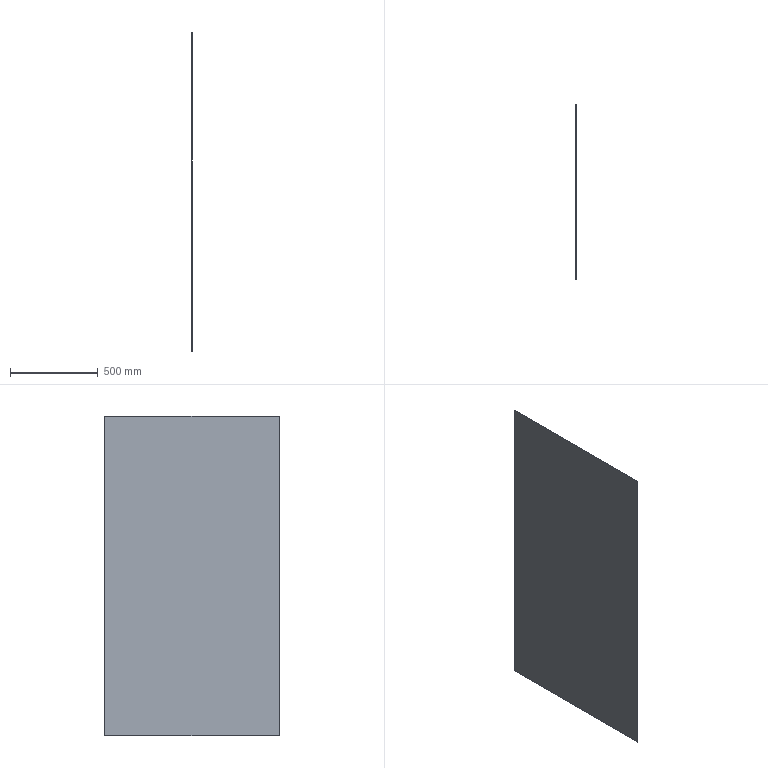Component | SolidWorks | BackPlate-3 | 1 solid | 9 faces | box 1.5 x 997 x 1820 mm | volume 2719006 mm3 | plane 9
STEP:
#1=COLOUR_RGB('',0.7922,0.8196,0.9333);
#2=FILL_AREA_STYLE_COLOUR('',#1);
#3=FILL_AREA_STYLE('',(#2));
#4=SURFACE_STYLE_FILL_AREA(#3);
#5=SURFACE_SIDE_STYLE('',(#4));
#6=SURFACE_STYLE_USAGE(.BOTH.,#5);
#7=PRESENTATION_STYLE_ASSIGNMENT((#6));
#8=CARTESIAN_POINT('',(19.524,29.311,66.594));
#9=VERTEX_POINT('',#8);
#10=CARTESIAN_POINT('',(19.508,29.311,66.594));
#11=VERTEX_POINT('',#10);
#12=CARTESIAN_POINT('',(19.567,29.311,66.594));
#13=DIRECTION('',(-1.,0.,0.));
#14=VECTOR('',#13,39.37);
#15=LINE('',#12,#14);
#16=EDGE_CURVE('',#9,#11,#15,.T.);
#17=ORIENTED_EDGE('',*,*,#16,.F.);
#18=CARTESIAN_POINT('',(19.524,29.311,-5.059));
#19=VERTEX_POINT('',#18);
#20=CARTESIAN_POINT('',(19.524,29.311,-5.059));
#21=DIRECTION('',(0.,0.,-1.));
#22=VECTOR('',#21,39.37);
#23=LINE('',#20,#22);
#24=EDGE_CURVE('',#9,#19,#23,.T.);
#25=ORIENTED_EDGE('',*,*,#24,.T.);
#26=CARTESIAN_POINT('',(19.508,29.311,-5.059));
#27=VERTEX_POINT('',#26);
#28=CARTESIAN_POINT('',(19.567,29.311,-5.059));
#29=DIRECTION('',(-1.,0.,0.));
#30=VECTOR('',#29,39.37);
#31=LINE('',#28,#30);
#32=EDGE_CURVE('',#19,#27,#31,.T.);
#33=ORIENTED_EDGE('',*,*,#32,.T.);
#34=CARTESIAN_POINT('',(19.508,29.311,-5.059));
#35=DIRECTION('',(0.,0.,-1.));
#36=VECTOR('',#35,39.37);
#37=LINE('',#34,#36);
#38=EDGE_CURVE('',#11,#27,#37,.T.);
#39=ORIENTED_EDGE('',*,*,#38,.F.);
#40=EDGE_LOOP('',(#17,#25,#33,#39));
#41=FACE_OUTER_BOUND('',#40,.T.);
#42=CARTESIAN_POINT('',(19.567,29.311,-5.059));
#43=DIRECTION('',(0.,1.,0.));
#44=DIRECTION('',(0.,0.,-1.));
#45=AXIS2_PLACEMENT_3D('',#42,#43,#44);
#46=PLANE('',#45);
#47=ADVANCED_FACE('',(#41),#46,.T.);
#48=CARTESIAN_POINT('',(19.524,-9.941,66.594));
#49=VERTEX_POINT('',#48);
#50=CARTESIAN_POINT('',(19.508,-9.941,66.594));
#51=VERTEX_POINT('',#50);
#52=CARTESIAN_POINT('',(19.567,-9.941,66.594));
#53=DIRECTION('',(-1.,0.,0.));
#54=VECTOR('',#53,39.37);
#55=LINE('',#52,#54);
#56=EDGE_CURVE('',#49,#51,#55,.T.);
#57=ORIENTED_EDGE('',*,*,#56,.F.);
#58=CARTESIAN_POINT('',(19.524,29.311,66.594));
#59=DIRECTION('',(0.,1.,0.));
#60=VECTOR('',#59,39.37);
#61=LINE('',#58,#60);
#62=EDGE_CURVE('',#49,#9,#61,.T.);
#63=ORIENTED_EDGE('',*,*,#62,.T.);
#64=ORIENTED_EDGE('',*,*,#16,.T.);
#65=CARTESIAN_POINT('',(19.508,-9.941,66.594));
#66=DIRECTION('',(0.,1.,0.));
#67=VECTOR('',#66,39.37);
#68=LINE('',#65,#67);
#69=EDGE_CURVE('',#51,#11,#68,.T.);
#70=ORIENTED_EDGE('',*,*,#69,.F.);
#71=EDGE_LOOP('',(#57,#63,#64,#70));
#72=FACE_OUTER_BOUND('',#71,.T.);
#73=CARTESIAN_POINT('',(19.567,-9.941,66.594));
#74=DIRECTION('',(0.,-0.,1.));
#75=DIRECTION('',(1.,-0.,-0.));
#76=AXIS2_PLACEMENT_3D('',#73,#74,#75);
#77=PLANE('',#76);
#78=ADVANCED_FACE('',(#72),#77,.T.);
#79=CARTESIAN_POINT('',(19.524,-9.941,-5.059));
#80=VERTEX_POINT('',#79);
#81=CARTESIAN_POINT('',(19.508,-9.941,-5.059));
#82=VERTEX_POINT('',#81);
#83=CARTESIAN_POINT('',(19.567,-9.941,-5.059));
#84=DIRECTION('',(-1.,0.,0.));
#85=VECTOR('',#84,39.37);
#86=LINE('',#83,#85);
#87=EDGE_CURVE('',#80,#82,#86,.T.);
#88=ORIENTED_EDGE('',*,*,#87,.F.);
#89=CARTESIAN_POINT('',(19.524,-9.941,66.594));
#90=DIRECTION('',(-0.,-0.,1.));
#91=VECTOR('',#90,39.37);
#92=LINE('',#89,#91);
#93=EDGE_CURVE('',#80,#49,#92,.T.);
#94=ORIENTED_EDGE('',*,*,#93,.T.);
#95=ORIENTED_EDGE('',*,*,#56,.T.);
#96=CARTESIAN_POINT('',(19.508,-9.941,-5.059));
#97=DIRECTION('',(-0.,-0.,1.));
#98=VECTOR('',#97,39.37);
#99=LINE('',#96,#98);
#100=EDGE_CURVE('',#82,#51,#99,.T.);
#101=ORIENTED_EDGE('',*,*,#100,.F.);
#102=EDGE_LOOP('',(#88,#94,#95,#101));
#103=FACE_OUTER_BOUND('',#102,.T.);
#104=CARTESIAN_POINT('',(19.567,-9.941,-5.059));
#105=DIRECTION('',(-0.,-1.,-0.));
#106=DIRECTION('',(-0.,-0.,1.));
#107=AXIS2_PLACEMENT_3D('',#104,#105,#106);
#108=PLANE('',#107);
#109=ADVANCED_FACE('',(#103),#108,.T.);
#110=ORIENTED_EDGE('',*,*,#32,.F.);
#111=CARTESIAN_POINT('',(19.567,29.268,-5.059));
#112=VERTEX_POINT('',#111);
#113=CARTESIAN_POINT('',(39.171,9.663,-5.059));
#114=DIRECTION('',(0.7071,-0.7071,-0.));
#115=VECTOR('',#114,39.37);
#116=LINE('',#113,#115);
#117=EDGE_CURVE('',#19,#112,#116,.T.);
#118=ORIENTED_EDGE('',*,*,#117,.T.);
#119=CARTESIAN_POINT('',(19.567,-9.898,-5.059));
#120=VERTEX_POINT('',#119);
#121=CARTESIAN_POINT('',(19.567,-9.941,-5.059));
#122=DIRECTION('',(-0.,-1.,-0.));
#123=VECTOR('',#122,39.37);
#124=LINE('',#121,#123);
#125=EDGE_CURVE('',#112,#120,#124,.T.);
#126=ORIENTED_EDGE('',*,*,#125,.T.);
#127=CARTESIAN_POINT('',(19.545,-9.919,-5.059));
#128=DIRECTION('',(-0.7071,-0.7071,-0.));
#129=VECTOR('',#128,39.37);
#130=LINE('',#127,#129);
#131=EDGE_CURVE('',#120,#80,#130,.T.);
#132=ORIENTED_EDGE('',*,*,#131,.T.);
#133=ORIENTED_EDGE('',*,*,#87,.T.);
#134=CARTESIAN_POINT('',(19.508,-9.941,-5.059));
#135=DIRECTION('',(-0.,-1.,-0.));
#136=VECTOR('',#135,39.37);
#137=LINE('',#134,#136);
#138=EDGE_CURVE('',#27,#82,#137,.T.);
#139=ORIENTED_EDGE('',*,*,#138,.F.);
#140=EDGE_LOOP('',(#110,#118,#126,#132,#133,#139));
#141=FACE_OUTER_BOUND('',#140,.T.);
#142=CARTESIAN_POINT('',(19.567,-9.941,-5.059));
#143=DIRECTION('',(-0.,0.,-1.));
#144=DIRECTION('',(-1.,0.,0.));
#145=AXIS2_PLACEMENT_3D('',#142,#143,#144);
#146=PLANE('',#145);
#147=ADVANCED_FACE('',(#141),#146,.T.);
#148=ORIENTED_EDGE('',*,*,#125,.F.);
#149=CARTESIAN_POINT('',(19.567,29.268,66.551));
#150=VERTEX_POINT('',#149);
#151=CARTESIAN_POINT('',(19.567,29.268,66.594));
#152=DIRECTION('',(-0.,-0.,1.));
#153=VECTOR('',#152,39.37);
#154=LINE('',#151,#153);
#155=EDGE_CURVE('',#112,#150,#154,.T.);
#156=ORIENTED_EDGE('',*,*,#155,.T.);
#157=CARTESIAN_POINT('',(19.567,-9.898,66.551));
#158=VERTEX_POINT('',#157);
#159=CARTESIAN_POINT('',(19.567,-9.941,66.551));
#160=DIRECTION('',(-0.,-1.,-0.));
#161=VECTOR('',#160,39.37);
#162=LINE('',#159,#161);
#163=EDGE_CURVE('',#150,#158,#162,.T.);
#164=ORIENTED_EDGE('',*,*,#163,.T.);
#165=CARTESIAN_POINT('',(19.567,-9.898,-5.059));
#166=DIRECTION('',(0.,0.,-1.));
#167=VECTOR('',#166,39.37);
#168=LINE('',#165,#167);
#169=EDGE_CURVE('',#158,#120,#168,.T.);
#170=ORIENTED_EDGE('',*,*,#169,.T.);
#171=EDGE_LOOP('',(#148,#156,#164,#170));
#172=FACE_OUTER_BOUND('',#171,.T.);
#173=CARTESIAN_POINT('',(19.567,9.685,30.768));
#174=DIRECTION('',(-1.,0.,0.));
#175=DIRECTION('',(0.,1.,0.));
#176=AXIS2_PLACEMENT_3D('',#173,#174,#175);
#177=PLANE('',#176);
#178=ADVANCED_FACE('',(#172),#177,.F.);
#179=ORIENTED_EDGE('',*,*,#38,.T.);
#180=ORIENTED_EDGE('',*,*,#138,.T.);
#181=ORIENTED_EDGE('',*,*,#100,.T.);
#182=ORIENTED_EDGE('',*,*,#69,.T.);
#183=EDGE_LOOP('',(#179,#180,#181,#182));
#184=FACE_OUTER_BOUND('',#183,.T.);
#185=CARTESIAN_POINT('',(19.508,9.685,30.768));
#186=DIRECTION('',(-1.,0.,0.));
#187=DIRECTION('',(0.,1.,0.));
#188=AXIS2_PLACEMENT_3D('',#185,#186,#187);
#189=PLANE('',#188);
#190=ADVANCED_FACE('',(#184),#189,.T.);
#191=ORIENTED_EDGE('',*,*,#131,.F.);
#192=ORIENTED_EDGE('',*,*,#169,.F.);
#193=CARTESIAN_POINT('',(19.524,-9.941,66.594));
#194=DIRECTION('',(0.5774,0.5774,-0.5774));
#195=VECTOR('',#194,39.37);
#196=LINE('',#193,#195);
#197=EDGE_CURVE('',#49,#158,#196,.T.);
#198=ORIENTED_EDGE('',*,*,#197,.F.);
#199=ORIENTED_EDGE('',*,*,#93,.F.);
#200=EDGE_LOOP('',(#191,#192,#198,#199));
#201=FACE_OUTER_BOUND('',#200,.T.);
#202=CARTESIAN_POINT('',(19.524,-9.941,-5.059));
#203=DIRECTION('',(0.7071,-0.7071,-0.));
#204=DIRECTION('',(0.,0.,-1.));
#205=AXIS2_PLACEMENT_3D('',#202,#203,#204);
#206=PLANE('',#205);
#207=ADVANCED_FACE('',(#201),#206,.T.);
#208=ORIENTED_EDGE('',*,*,#197,.T.);
#209=ORIENTED_EDGE('',*,*,#163,.F.);
#210=CARTESIAN_POINT('',(32.608,16.227,53.51));
#211=DIRECTION('',(0.5774,-0.5774,-0.5774));
#212=VECTOR('',#211,39.37);
#213=LINE('',#210,#212);
#214=EDGE_CURVE('',#9,#150,#213,.T.);
#215=ORIENTED_EDGE('',*,*,#214,.F.);
#216=ORIENTED_EDGE('',*,*,#62,.F.);
#217=EDGE_LOOP('',(#208,#209,#215,#216));
#218=FACE_OUTER_BOUND('',#217,.T.);
#219=CARTESIAN_POINT('',(19.524,-9.941,66.594));
#220=DIRECTION('',(0.7071,-0.,0.7071));
#221=DIRECTION('',(-0.,-1.,-0.));
#222=AXIS2_PLACEMENT_3D('',#219,#220,#221);
#223=PLANE('',#222);
#224=ADVANCED_FACE('',(#218),#223,.T.);
#225=ORIENTED_EDGE('',*,*,#214,.T.);
#226=ORIENTED_EDGE('',*,*,#155,.F.);
#227=ORIENTED_EDGE('',*,*,#117,.F.);
#228=ORIENTED_EDGE('',*,*,#24,.F.);
#229=EDGE_LOOP('',(#225,#226,#227,#228));
#230=FACE_OUTER_BOUND('',#229,.T.);
#231=CARTESIAN_POINT('',(19.524,29.311,-5.059));
#232=DIRECTION('',(0.7071,0.7071,0.));
#233=DIRECTION('',(-0.,-0.,1.));
#234=AXIS2_PLACEMENT_3D('',#231,#232,#233);
#235=PLANE('',#234);
#236=ADVANCED_FACE('',(#230),#235,.T.);
#237=CLOSED_SHELL('',(#47,#78,#109,#147,#178,#190,#207,#224,#236));
#238=MANIFOLD_SOLID_BREP('',#237);
#239=STYLED_ITEM('',(#7),#238);
#240=(LENGTH_UNIT()NAMED_UNIT(*)SI_UNIT($,.METRE.));
#241=LENGTH_MEASURE_WITH_UNIT(LENGTH_MEASURE(0.0254),#240);
#242=DIMENSIONAL_EXPONENTS(1.,0.,0.,0.,0.,0.,0.);
#243=(CONVERSION_BASED_UNIT('',#241)LENGTH_UNIT()NAMED_UNIT(#242));
#244=UNCERTAINTY_MEASURE_WITH_UNIT(LENGTH_MEASURE(0.00001),#243,'','');
#245=(NAMED_UNIT(*)PLANE_ANGLE_UNIT()SI_UNIT($,.RADIAN.));
#246=(NAMED_UNIT(*)SI_UNIT($,.STERADIAN.)SOLID_ANGLE_UNIT());
#247=(GEOMETRIC_REPRESENTATION_CONTEXT(3)GLOBAL_UNCERTAINTY_ASSIGNED_CONTEXT((#244))GLOBAL_UNIT_ASSIGNED_CONTEXT((#243,#245,#246))REPRESENTATION_CONTEXT('',''));
#248=MECHANICAL_DESIGN_GEOMETRIC_PRESENTATION_REPRESENTATION('',(#239),#247);
#249=PRESENTATION_LAYER_ASSIGNMENT('','',(#239));
#250=CARTESIAN_POINT('',(0.,0.,0.));
#251=DIRECTION('',(0.,0.,1.));
#252=DIRECTION('',(1.,0.,0.));
#253=AXIS2_PLACEMENT_3D('',#250,#251,#252);
#254=(LENGTH_UNIT()NAMED_UNIT(*)SI_UNIT($,.METRE.));
#255=LENGTH_MEASURE_WITH_UNIT(LENGTH_MEASURE(0.0254),#254);
#256=DIMENSIONAL_EXPONENTS(1.,0.,0.,0.,0.,0.,0.);
#257=(CONVERSION_BASED_UNIT('',#255)LENGTH_UNIT()NAMED_UNIT(#256));
#258=UNCERTAINTY_MEASURE_WITH_UNIT(LENGTH_MEASURE(0.00001),#257,'','');
#259=(NAMED_UNIT(*)PLANE_ANGLE_UNIT()SI_UNIT($,.RADIAN.));
#260=(NAMED_UNIT(*)SI_UNIT($,.STERADIAN.)SOLID_ANGLE_UNIT());
#261=(GEOMETRIC_REPRESENTATION_CONTEXT(3)GLOBAL_UNCERTAINTY_ASSIGNED_CONTEXT((#258))GLOBAL_UNIT_ASSIGNED_CONTEXT((#257,#259,#260))REPRESENTATION_CONTEXT('',''));
#262=ADVANCED_BREP_SHAPE_REPRESENTATION('',(#238,#253),#261);